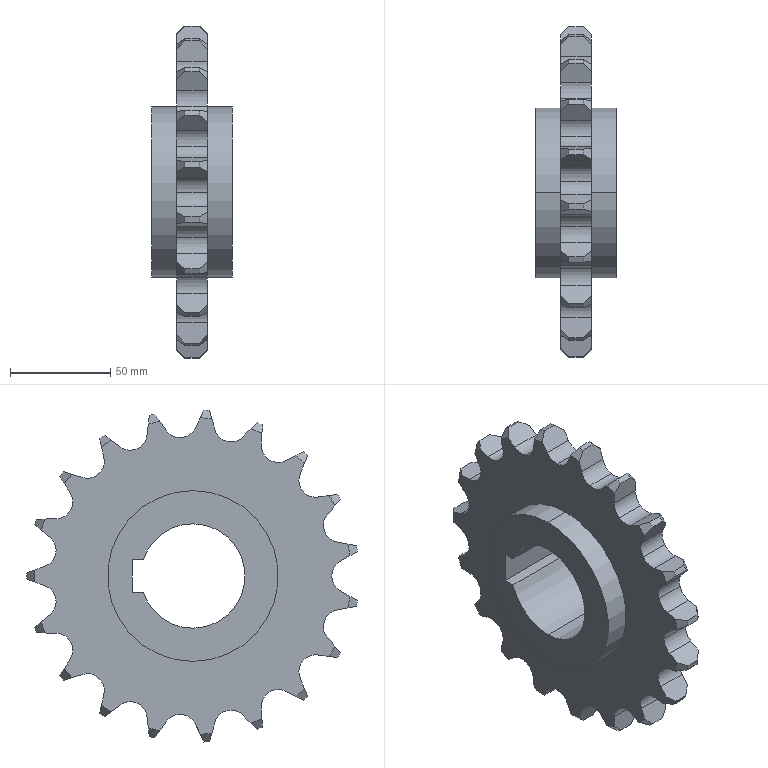Component | SolidWorks | 19ToothSprocket-1 | 1 solid | 153 faces | box 40 x 164.79 x 165.34 mm | volume 312024 mm3 | cylinder 70 | plane 45 | cone 38 | commonest cylinder face diameters 15.88 x44 165.7 x19 85 x4 52 x3
build123d program:
from build123d import *

# Parameters (mm, degrees)
SKETCH1_R           = 42.5
BOSS_EXTRUDE1_DEPTH = 20
SKETCH2_R           = 82.85
BOSS_EXTRUDE2_DEPTH = 7.5
CUT_EXTRUDE1_DEPTH  = 121.352
CIRPATTERN1_COUNT   = 19
CHAMFER1_SIZE       = 4


with BuildPart() as part:
    # Sketch1 → Boss-Extrude1 (new, symmetric)
    with BuildSketch(Plane.XY):
        Circle(SKETCH1_R)
        with BuildLine():
            Line((-8, 30.3), (8, 30.3))
            Line((8, 30.3), (8, 24.739))
            ThreePointArc((8, 24.739), (0, -26), (-8, 24.739))
            Line((-8, 24.739), (-8, 30.3))
        make_face(mode=Mode.SUBTRACT)
    extrude(amount=BOSS_EXTRUDE1_DEPTH, both=True)

    # Sketch2 → Boss-Extrude2 (add, symmetric)
    with BuildSketch(Plane.XY):
        Circle(SKETCH2_R)
        with BuildLine():
            Line((-8, 30.3), (-8, 24.739))
            ThreePointArc((-8, 24.739), (0, -26), (8, 24.739))
            Line((8, 24.739), (8, 30.3))
            Line((8, 30.3), (-8, 30.3))
        make_face(mode=Mode.SUBTRACT)
    extrude(amount=BOSS_EXTRUDE2_DEPTH, both=True)

    # Sketch3 → Cut-Extrude1 (cut, through all)
    with BuildSketch(Plane.XY.offset(7.5)):
        with BuildLine():
            Line((18.589, 71.123), (25.017, 78.983))
            ThreePointArc((25.017, 78.983), (13.36, 81.766), (1.424, 82.838))
            Line((1.424, 82.838), (5.016, 73.341))
            ThreePointArc((5.016, 73.341), (11.162, 68.314), (18.589, 71.123))
        make_face()
        with BuildLine():
            Line((-1.424, 82.838), (-5.016, 73.341))
            ThreePointArc((-5.016, 73.341), (-11.162, 68.314), (-18.589, 71.123))
            Line((-18.589, 71.123), (-25.017, 78.983))
            ThreePointArc((-25.017, 78.983), (-13.36, 81.766), (-1.424, 82.838))
        make_face()
    cut_extrude1 = extrude(amount=-CUT_EXTRUDE1_DEPTH, mode=Mode.SUBTRACT)

    # CirPattern1: Cut-Extrude1 ×19 about axis
    cirpattern1_axis = Axis((0, 0, 0), (0, 0, 1))
    for i in range(1, CIRPATTERN1_COUNT):
        add(cut_extrude1.rotate(cirpattern1_axis, i * 360 / CIRPATTERN1_COUNT), mode=Mode.SUBTRACT)

    # Chamfer1
    chamfer1_edges = [part.edges().sort_by_distance(p)[0] for p in [
        (50.888, 65.38, -7.5),
        (50.888, 65.38, 7.5),
        (69.359, 45.315, -7.5),
        (69.359, 45.315, 7.5),
        (80.315, 20.338, -7.5),
        (80.315, 20.338, 7.5),
        (82.567, -6.842, -7.5),
        (82.567, -6.842, 7.5),
        (75.872, -33.28, -7.5),
        (75.872, -33.28, 7.5),
        (60.955, -56.113, -7.5),
        (60.955, -56.113, 7.5),
        (39.432, -72.864, -7.5),
        (39.432, -72.864, 7.5),
        (13.637, -81.72, -7.5),
        (13.637, -81.72, 7.5),
        (-13.637, -81.72, -7.5),
        (-13.637, -81.72, 7.5),
        (-39.432, -72.864, -7.5),
        (-39.432, -72.864, 7.5),
        (-60.955, -56.113, -7.5),
        (-60.955, -56.113, 7.5),
        (-75.872, -33.28, -7.5),
        (-75.872, -33.28, 7.5),
        (-82.567, -6.842, -7.5),
        (-82.567, -6.842, 7.5),
        (-80.315, 20.338, -7.5),
        (-80.315, 20.338, 7.5),
        (0, 82.85, 7.5),
        (-69.359, 45.315, -7.5),
        (0, 82.85, -7.5),
        (-69.359, 45.315, 7.5),
        (-50.888, 65.38, -7.5),
        (-50.888, 65.38, 7.5),
        (-26.901, 78.361, -7.5),
        (-26.901, 78.361, 7.5),
        (26.901, 78.361, -7.5),
        (26.901, 78.361, 7.5),
    ]]
    chamfer(chamfer1_edges, length=CHAMFER1_SIZE)


solid = part.part

# Placed as in the assembly
solid = solid.moved(Location((-771.197, 34.532, 0), (0, 90, 0)))